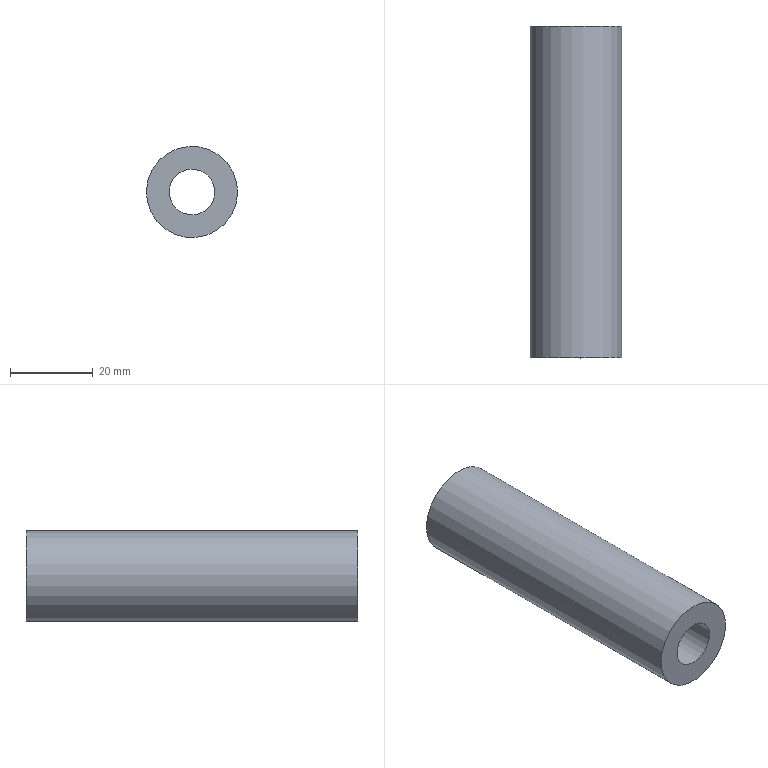Component | NX | PISTON_PIN | 1 solid | 4 faces | box 22 x 80 x 22 mm | volume 22808 mm3 | cylinder 2 | plane 2 | commonest cylinder face diameters 22 x1 11 x1
STEP:
#1=CARTESIAN_POINT('',(0.,0.,0.));
#2=DIRECTION('',(0.,0.,1.));
#3=DIRECTION('',(1.,0.,0.));
#4=AXIS2_PLACEMENT_3D('',#1,#2,#3);
#5=CARTESIAN_POINT('',(80.393,-40.,216.606));
#6=VERTEX_POINT('',#5);
#7=CARTESIAN_POINT('',(69.635,-40.,214.314));
#8=DIRECTION('',(0.,-1.,0.));
#9=DIRECTION('',(0.978,0.,0.2084));
#10=AXIS2_PLACEMENT_3D('',#7,#8,#9);
#11=CIRCLE('',#10,11.);
#12=CARTESIAN_POINT('',(69.635,-40.,214.314));
#13=DIRECTION('',(0.,1.,0.));
#14=DIRECTION('',(-0.978,0.,-0.2084));
#15=AXIS2_PLACEMENT_3D('',#12,#13,#14);
#16=CYLINDRICAL_SURFACE('',#15,11.);
#17=CARTESIAN_POINT('',(9.425,0.));
#18=DIRECTION('',(-1.,0.));
#19=VECTOR('',#18,1.);
#20=LINE('',#17,#19);
#21=(GEOMETRIC_REPRESENTATION_CONTEXT(2)PARAMETRIC_REPRESENTATION_CONTEXT()REPRESENTATION_CONTEXT('',''));
#22=DEFINITIONAL_REPRESENTATION('',(#20),#21);
#23=PCURVE('',#16,#22);
#24=CARTESIAN_POINT('',(69.635,-40.,214.314));
#25=DIRECTION('',(0.,-1.,0.));
#26=DIRECTION('',(0.978,0.,0.2084));
#27=AXIS2_PLACEMENT_3D('',#24,#25,#26);
#28=PLANE('',#27);
#29=CARTESIAN_POINT('',(0.,0.));
#30=DIRECTION('',(1.,-0.));
#31=AXIS2_PLACEMENT_2D('',#29,#30);
#32=CIRCLE('',#31,11.);
#33=(GEOMETRIC_REPRESENTATION_CONTEXT(2)PARAMETRIC_REPRESENTATION_CONTEXT()REPRESENTATION_CONTEXT('',''));
#34=DEFINITIONAL_REPRESENTATION('',(#32),#33);
#35=PCURVE('',#28,#34);
#36=SURFACE_CURVE('',#11,(#23,#35),.PCURVE_S1.);
#37=EDGE_CURVE('',#6,#6,#36,.T.);
#38=ORIENTED_EDGE('',*,*,#37,.F.);
#39=CARTESIAN_POINT('',(80.393,40.,216.606));
#40=VERTEX_POINT('',#39);
#41=CARTESIAN_POINT('',(80.393,-40.,216.606));
#42=CARTESIAN_POINT('',(80.393,40.,216.606));
#43=B_SPLINE_CURVE_WITH_KNOTS('',1,(#41,#42),.UNSPECIFIED.,.F.,.F.,(2,2),(0.,80.),.PIECEWISE_BEZIER_KNOTS.);
#44=CARTESIAN_POINT('',(9.425,0.));
#45=DIRECTION('',(0.,1.));
#46=VECTOR('',#45,1.);
#47=LINE('',#44,#46);
#48=(GEOMETRIC_REPRESENTATION_CONTEXT(2)PARAMETRIC_REPRESENTATION_CONTEXT()REPRESENTATION_CONTEXT('',''));
#49=DEFINITIONAL_REPRESENTATION('',(#47),#48);
#50=PCURVE('',#16,#49);
#51=CARTESIAN_POINT('',(3.142,0.));
#52=DIRECTION('',(0.,1.));
#53=VECTOR('',#52,1.);
#54=LINE('',#51,#53);
#55=(GEOMETRIC_REPRESENTATION_CONTEXT(2)PARAMETRIC_REPRESENTATION_CONTEXT()REPRESENTATION_CONTEXT('',''));
#56=DEFINITIONAL_REPRESENTATION('',(#54),#55);
#57=PCURVE('',#16,#56);
#58=SEAM_CURVE('',#43,(#50,#57),.PCURVE_S1.);
#59=EDGE_CURVE('',#6,#40,#58,.T.);
#60=ORIENTED_EDGE('',*,*,#59,.T.);
#61=CARTESIAN_POINT('',(69.635,40.,214.314));
#62=DIRECTION('',(0.,-1.,0.));
#63=DIRECTION('',(0.978,0.,0.2084));
#64=AXIS2_PLACEMENT_3D('',#61,#62,#63);
#65=CIRCLE('',#64,11.);
#66=CARTESIAN_POINT('',(9.425,80.));
#67=DIRECTION('',(-1.,0.));
#68=VECTOR('',#67,1.);
#69=LINE('',#66,#68);
#70=(GEOMETRIC_REPRESENTATION_CONTEXT(2)PARAMETRIC_REPRESENTATION_CONTEXT()REPRESENTATION_CONTEXT('',''));
#71=DEFINITIONAL_REPRESENTATION('',(#69),#70);
#72=PCURVE('',#16,#71);
#73=CARTESIAN_POINT('',(69.635,40.,214.314));
#74=DIRECTION('',(0.,-1.,0.));
#75=DIRECTION('',(0.978,0.,0.2084));
#76=AXIS2_PLACEMENT_3D('',#73,#74,#75);
#77=PLANE('',#76);
#78=CARTESIAN_POINT('',(0.,0.));
#79=DIRECTION('',(1.,-0.));
#80=AXIS2_PLACEMENT_2D('',#78,#79);
#81=CIRCLE('',#80,11.);
#82=(GEOMETRIC_REPRESENTATION_CONTEXT(2)PARAMETRIC_REPRESENTATION_CONTEXT()REPRESENTATION_CONTEXT('',''));
#83=DEFINITIONAL_REPRESENTATION('',(#81),#82);
#84=PCURVE('',#77,#83);
#85=SURFACE_CURVE('',#65,(#72,#84),.PCURVE_S1.);
#86=EDGE_CURVE('',#40,#40,#85,.T.);
#87=ORIENTED_EDGE('',*,*,#86,.T.);
#88=ORIENTED_EDGE('',*,*,#59,.F.);
#89=EDGE_LOOP('',(#38,#60,#87,#88));
#90=FACE_BOUND('',#89,.T.);
#91=ADVANCED_FACE('',(#90),#16,.T.);
#92=CARTESIAN_POINT('',(75.014,-40.,215.46));
#93=VERTEX_POINT('',#92);
#94=CARTESIAN_POINT('',(69.635,-40.,214.314));
#95=DIRECTION('',(0.,-1.,0.));
#96=DIRECTION('',(0.978,0.,0.2084));
#97=AXIS2_PLACEMENT_3D('',#94,#95,#96);
#98=CIRCLE('',#97,5.5);
#99=CARTESIAN_POINT('',(69.635,-40.,214.314));
#100=DIRECTION('',(0.,1.,0.));
#101=DIRECTION('',(-0.978,0.,-0.2084));
#102=AXIS2_PLACEMENT_3D('',#99,#100,#101);
#103=CYLINDRICAL_SURFACE('',#102,5.5);
#104=CARTESIAN_POINT('',(9.425,0.));
#105=DIRECTION('',(-1.,0.));
#106=VECTOR('',#105,1.);
#107=LINE('',#104,#106);
#108=(GEOMETRIC_REPRESENTATION_CONTEXT(2)PARAMETRIC_REPRESENTATION_CONTEXT()REPRESENTATION_CONTEXT('',''));
#109=DEFINITIONAL_REPRESENTATION('',(#107),#108);
#110=PCURVE('',#103,#109);
#111=CARTESIAN_POINT('',(0.,0.));
#112=DIRECTION('',(1.,0.));
#113=AXIS2_PLACEMENT_2D('',#111,#112);
#114=CIRCLE('',#113,5.5);
#115=(GEOMETRIC_REPRESENTATION_CONTEXT(2)PARAMETRIC_REPRESENTATION_CONTEXT()REPRESENTATION_CONTEXT('',''));
#116=DEFINITIONAL_REPRESENTATION('',(#114),#115);
#117=PCURVE('',#28,#116);
#118=SURFACE_CURVE('',#98,(#110,#117),.PCURVE_S1.);
#119=EDGE_CURVE('',#93,#93,#118,.T.);
#120=ORIENTED_EDGE('',*,*,#119,.F.);
#121=CARTESIAN_POINT('',(75.014,40.,215.46));
#122=VERTEX_POINT('',#121);
#123=CARTESIAN_POINT('',(75.014,-40.,215.46));
#124=CARTESIAN_POINT('',(75.014,40.,215.46));
#125=B_SPLINE_CURVE_WITH_KNOTS('',1,(#123,#124),.UNSPECIFIED.,.F.,.F.,(2,2),(0.,80.),.PIECEWISE_BEZIER_KNOTS.);
#126=CARTESIAN_POINT('',(9.425,0.));
#127=DIRECTION('',(0.,1.));
#128=VECTOR('',#127,1.);
#129=LINE('',#126,#128);
#130=(GEOMETRIC_REPRESENTATION_CONTEXT(2)PARAMETRIC_REPRESENTATION_CONTEXT()REPRESENTATION_CONTEXT('',''));
#131=DEFINITIONAL_REPRESENTATION('',(#129),#130);
#132=PCURVE('',#103,#131);
#133=CARTESIAN_POINT('',(3.142,0.));
#134=DIRECTION('',(0.,1.));
#135=VECTOR('',#134,1.);
#136=LINE('',#133,#135);
#137=(GEOMETRIC_REPRESENTATION_CONTEXT(2)PARAMETRIC_REPRESENTATION_CONTEXT()REPRESENTATION_CONTEXT('',''));
#138=DEFINITIONAL_REPRESENTATION('',(#136),#137);
#139=PCURVE('',#103,#138);
#140=SEAM_CURVE('',#125,(#132,#139),.PCURVE_S1.);
#141=EDGE_CURVE('',#93,#122,#140,.T.);
#142=ORIENTED_EDGE('',*,*,#141,.T.);
#143=CARTESIAN_POINT('',(69.635,40.,214.314));
#144=DIRECTION('',(0.,-1.,0.));
#145=DIRECTION('',(0.978,0.,0.2084));
#146=AXIS2_PLACEMENT_3D('',#143,#144,#145);
#147=CIRCLE('',#146,5.5);
#148=CARTESIAN_POINT('',(9.425,80.));
#149=DIRECTION('',(-1.,0.));
#150=VECTOR('',#149,1.);
#151=LINE('',#148,#150);
#152=(GEOMETRIC_REPRESENTATION_CONTEXT(2)PARAMETRIC_REPRESENTATION_CONTEXT()REPRESENTATION_CONTEXT('',''));
#153=DEFINITIONAL_REPRESENTATION('',(#151),#152);
#154=PCURVE('',#103,#153);
#155=CARTESIAN_POINT('',(0.,0.));
#156=DIRECTION('',(1.,0.));
#157=AXIS2_PLACEMENT_2D('',#155,#156);
#158=CIRCLE('',#157,5.5);
#159=(GEOMETRIC_REPRESENTATION_CONTEXT(2)PARAMETRIC_REPRESENTATION_CONTEXT()REPRESENTATION_CONTEXT('',''));
#160=DEFINITIONAL_REPRESENTATION('',(#158),#159);
#161=PCURVE('',#77,#160);
#162=SURFACE_CURVE('',#147,(#154,#161),.PCURVE_S1.);
#163=EDGE_CURVE('',#122,#122,#162,.T.);
#164=ORIENTED_EDGE('',*,*,#163,.T.);
#165=ORIENTED_EDGE('',*,*,#141,.F.);
#166=EDGE_LOOP('',(#120,#142,#164,#165));
#167=FACE_BOUND('',#166,.F.);
#168=ADVANCED_FACE('',(#167),#103,.F.);
#169=ORIENTED_EDGE('',*,*,#37,.T.);
#170=EDGE_LOOP('',(#169));
#171=FACE_BOUND('',#170,.T.);
#172=ORIENTED_EDGE('',*,*,#119,.F.);
#173=EDGE_LOOP('',(#172));
#174=FACE_BOUND('',#173,.T.);
#175=ADVANCED_FACE('',(#171,#174),#28,.T.);
#176=ORIENTED_EDGE('',*,*,#86,.F.);
#177=EDGE_LOOP('',(#176));
#178=FACE_BOUND('',#177,.T.);
#179=ORIENTED_EDGE('',*,*,#163,.T.);
#180=EDGE_LOOP('',(#179));
#181=FACE_BOUND('',#180,.T.);
#182=ADVANCED_FACE('',(#178,#181),#77,.F.);
#183=CLOSED_SHELL('',(#91,#168,#175,#182));
#184=MANIFOLD_SOLID_BREP('',#183);
#185=(LENGTH_UNIT()NAMED_UNIT(*)SI_UNIT(.MILLI.,.METRE.));
#186=UNCERTAINTY_MEASURE_WITH_UNIT(LENGTH_MEASURE(0.00001),#185,'','');
#187=(NAMED_UNIT(*)PLANE_ANGLE_UNIT()SI_UNIT($,.RADIAN.));
#188=(NAMED_UNIT(*)SI_UNIT($,.STERADIAN.)SOLID_ANGLE_UNIT());
#189=(GEOMETRIC_REPRESENTATION_CONTEXT(3)GLOBAL_UNCERTAINTY_ASSIGNED_CONTEXT((#186))GLOBAL_UNIT_ASSIGNED_CONTEXT((#185,#187,#188))REPRESENTATION_CONTEXT('',''));
#190=ADVANCED_BREP_SHAPE_REPRESENTATION('',(#4,#184),#189);